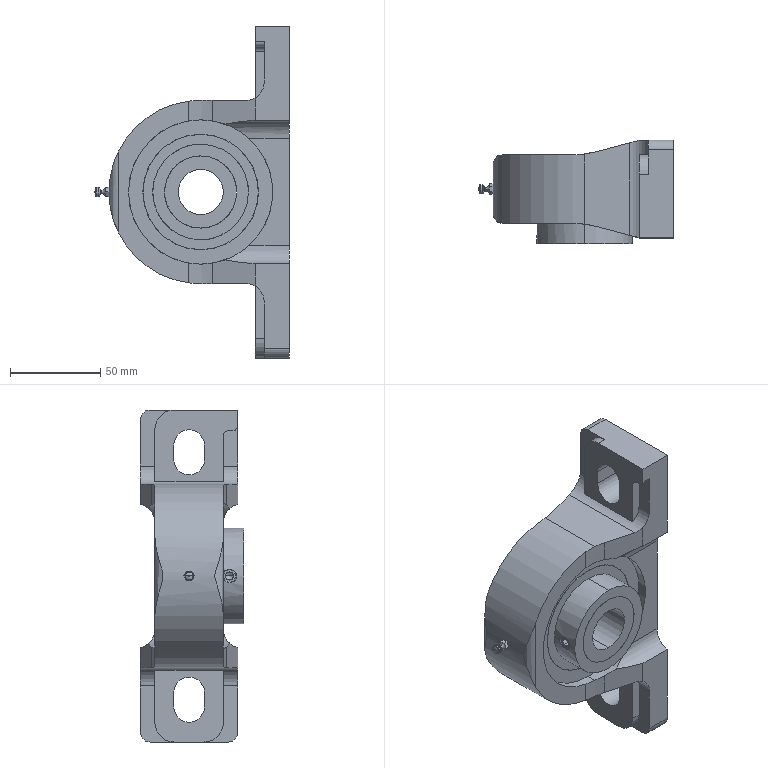Component | SolidWorks | RotatingBearingHousing-1 | 4 solids | 188 faces | volume 389061 mm3 | plane 76 | cylinder 57 | cone 39 | torus 16 | commonest cylinder face diameters 8 x8 6.917 x8 20.32 x6 101.6 x5 80 x4 40 x4 17 x4 10.8 x3 | material Plain Carbon Steel